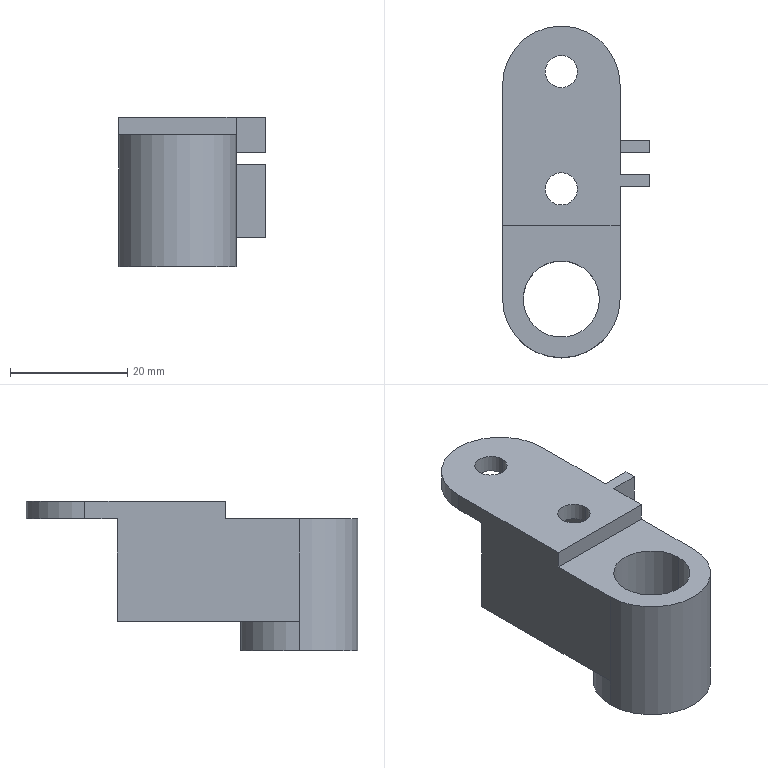Component | SolidWorks | CLS-MechanismAccessory1-1 | 1 solid | 31 faces | box 25 x 56.5 x 25.5 mm | volume 10042 mm3 | plane 21 | cylinder 10 | commonest cylinder face diameters 5.5 x4 20 x4 13 x2
STEP:
#1=COLOUR_RGB('',0.7922,0.8196,0.9333);
#2=FILL_AREA_STYLE_COLOUR('',#1);
#3=FILL_AREA_STYLE('',(#2));
#4=SURFACE_STYLE_FILL_AREA(#3);
#5=SURFACE_SIDE_STYLE('',(#4));
#6=SURFACE_STYLE_USAGE(.BOTH.,#5);
#7=PRESENTATION_STYLE_ASSIGNMENT((#6));
#8=CARTESIAN_POINT('',(-2.216,-0.1794,-0.1181));
#9=VERTEX_POINT('',#8);
#10=CARTESIAN_POINT('',(-2.432,-0.1794,-0.1181));
#11=VERTEX_POINT('',#10);
#12=CARTESIAN_POINT('',(-2.324,-0.1794,-0.1181));
#13=DIRECTION('',(-0.,0.,1.));
#14=DIRECTION('',(-1.,0.,0.));
#15=AXIS2_PLACEMENT_3D('',#12,#13,#14);
#16=CIRCLE('',#15,0.1083);
#17=EDGE_CURVE('',#9,#11,#16,.T.);
#18=ORIENTED_EDGE('',*,*,#17,.T.);
#19=CARTESIAN_POINT('',(-2.432,-0.1794,-0.2362));
#20=VERTEX_POINT('',#19);
#21=CARTESIAN_POINT('',(-2.432,-0.1794,-0.1181));
#22=DIRECTION('',(0.,-0.,-1.));
#23=VECTOR('',#22,39.37);
#24=LINE('',#21,#23);
#25=EDGE_CURVE('',#11,#20,#24,.T.);
#26=ORIENTED_EDGE('',*,*,#25,.T.);
#27=CARTESIAN_POINT('',(-2.216,-0.1794,-0.2362));
#28=VERTEX_POINT('',#27);
#29=CARTESIAN_POINT('',(-2.324,-0.1794,-0.2362));
#30=DIRECTION('',(0.,-0.,-1.));
#31=DIRECTION('',(1.,0.,0.));
#32=AXIS2_PLACEMENT_3D('',#29,#30,#31);
#33=CIRCLE('',#32,0.1083);
#34=EDGE_CURVE('',#20,#28,#33,.T.);
#35=ORIENTED_EDGE('',*,*,#34,.T.);
#36=CARTESIAN_POINT('',(-2.216,-0.1794,-0.1181));
#37=DIRECTION('',(0.,-0.,-1.));
#38=VECTOR('',#37,39.37);
#39=LINE('',#36,#38);
#40=EDGE_CURVE('',#9,#28,#39,.T.);
#41=ORIENTED_EDGE('',*,*,#40,.F.);
#42=EDGE_LOOP('',(#18,#26,#35,#41));
#43=FACE_OUTER_BOUND('',#42,.T.);
#44=CARTESIAN_POINT('',(-2.324,-0.1794,-0.1181));
#45=DIRECTION('',(0.,-0.,-1.));
#46=DIRECTION('',(1.,0.,0.));
#47=AXIS2_PLACEMENT_3D('',#44,#45,#46);
#48=CYLINDRICAL_SURFACE('',#47,0.1083);
#49=ADVANCED_FACE('',(#43),#48,.F.);
#50=CARTESIAN_POINT('',(-2.216,0.608,-0.1181));
#51=VERTEX_POINT('',#50);
#52=CARTESIAN_POINT('',(-2.432,0.608,-0.1181));
#53=VERTEX_POINT('',#52);
#54=CARTESIAN_POINT('',(-2.324,0.608,-0.1181));
#55=DIRECTION('',(-0.,0.,1.));
#56=DIRECTION('',(-1.,0.,0.));
#57=AXIS2_PLACEMENT_3D('',#54,#55,#56);
#58=CIRCLE('',#57,0.1083);
#59=EDGE_CURVE('',#51,#53,#58,.T.);
#60=ORIENTED_EDGE('',*,*,#59,.T.);
#61=CARTESIAN_POINT('',(-2.432,0.608,-0.2362));
#62=VERTEX_POINT('',#61);
#63=CARTESIAN_POINT('',(-2.432,0.608,-0.1181));
#64=DIRECTION('',(0.,-0.,-1.));
#65=VECTOR('',#64,39.37);
#66=LINE('',#63,#65);
#67=EDGE_CURVE('',#53,#62,#66,.T.);
#68=ORIENTED_EDGE('',*,*,#67,.T.);
#69=CARTESIAN_POINT('',(-2.216,0.608,-0.2362));
#70=VERTEX_POINT('',#69);
#71=CARTESIAN_POINT('',(-2.324,0.608,-0.2362));
#72=DIRECTION('',(0.,-0.,-1.));
#73=DIRECTION('',(1.,0.,0.));
#74=AXIS2_PLACEMENT_3D('',#71,#72,#73);
#75=CIRCLE('',#74,0.1083);
#76=EDGE_CURVE('',#62,#70,#75,.T.);
#77=ORIENTED_EDGE('',*,*,#76,.T.);
#78=CARTESIAN_POINT('',(-2.216,0.608,-0.1181));
#79=DIRECTION('',(0.,-0.,-1.));
#80=VECTOR('',#79,39.37);
#81=LINE('',#78,#80);
#82=EDGE_CURVE('',#51,#70,#81,.T.);
#83=ORIENTED_EDGE('',*,*,#82,.F.);
#84=EDGE_LOOP('',(#60,#68,#77,#83));
#85=FACE_OUTER_BOUND('',#84,.T.);
#86=CARTESIAN_POINT('',(-2.324,0.608,-0.1181));
#87=DIRECTION('',(0.,-0.,-1.));
#88=DIRECTION('',(1.,0.,0.));
#89=AXIS2_PLACEMENT_3D('',#86,#87,#88);
#90=CYLINDRICAL_SURFACE('',#89,0.1083);
#91=ADVANCED_FACE('',(#85),#90,.F.);
#92=CARTESIAN_POINT('',(-2.58,-0.9176,-0.2362));
#93=VERTEX_POINT('',#92);
#94=CARTESIAN_POINT('',(-2.068,-0.9176,-0.2362));
#95=VERTEX_POINT('',#94);
#96=CARTESIAN_POINT('',(-2.324,-0.9176,-0.2362));
#97=DIRECTION('',(0.,-0.,-1.));
#98=DIRECTION('',(1.,0.,0.));
#99=AXIS2_PLACEMENT_3D('',#96,#97,#98);
#100=CIRCLE('',#99,0.2559);
#101=EDGE_CURVE('',#93,#95,#100,.T.);
#102=ORIENTED_EDGE('',*,*,#101,.F.);
#103=CARTESIAN_POINT('',(-2.58,-0.9176,-1.122));
#104=VERTEX_POINT('',#103);
#105=CARTESIAN_POINT('',(-2.58,-0.9176,-0.2362));
#106=DIRECTION('',(0.,-0.,-1.));
#107=VECTOR('',#106,39.37);
#108=LINE('',#105,#107);
#109=EDGE_CURVE('',#93,#104,#108,.T.);
#110=ORIENTED_EDGE('',*,*,#109,.T.);
#111=CARTESIAN_POINT('',(-2.068,-0.9176,-1.122));
#112=VERTEX_POINT('',#111);
#113=CARTESIAN_POINT('',(-2.324,-0.9176,-1.122));
#114=DIRECTION('',(0.,-0.,-1.));
#115=DIRECTION('',(1.,0.,0.));
#116=AXIS2_PLACEMENT_3D('',#113,#114,#115);
#117=CIRCLE('',#116,0.2559);
#118=EDGE_CURVE('',#104,#112,#117,.T.);
#119=ORIENTED_EDGE('',*,*,#118,.T.);
#120=CARTESIAN_POINT('',(-2.068,-0.9176,-0.2362));
#121=DIRECTION('',(0.,-0.,-1.));
#122=VECTOR('',#121,39.37);
#123=LINE('',#120,#122);
#124=EDGE_CURVE('',#95,#112,#123,.T.);
#125=ORIENTED_EDGE('',*,*,#124,.F.);
#126=EDGE_LOOP('',(#102,#110,#119,#125));
#127=FACE_OUTER_BOUND('',#126,.T.);
#128=CARTESIAN_POINT('',(-2.324,-0.9176,-0.2362));
#129=DIRECTION('',(0.,-0.,-1.));
#130=DIRECTION('',(1.,0.,0.));
#131=AXIS2_PLACEMENT_3D('',#128,#129,#130);
#132=CYLINDRICAL_SURFACE('',#131,0.2559);
#133=ADVANCED_FACE('',(#127),#132,.F.);
#134=CARTESIAN_POINT('',(-1.93,-0.9176,-1.122));
#135=VERTEX_POINT('',#134);
#136=CARTESIAN_POINT('',(-2.718,-0.9176,-1.122));
#137=VERTEX_POINT('',#136);
#138=CARTESIAN_POINT('',(-2.324,-0.9176,-1.122));
#139=DIRECTION('',(0.,-0.,-1.));
#140=DIRECTION('',(1.,0.,0.));
#141=AXIS2_PLACEMENT_3D('',#138,#139,#140);
#142=CIRCLE('',#141,0.3937);
#143=EDGE_CURVE('',#135,#137,#142,.T.);
#144=ORIENTED_EDGE('',*,*,#143,.F.);
#145=CARTESIAN_POINT('',(-1.93,-0.9176,-0.9252));
#146=VERTEX_POINT('',#145);
#147=CARTESIAN_POINT('',(-1.93,-0.9176,-0.9252));
#148=DIRECTION('',(-0.,0.,1.));
#149=VECTOR('',#148,39.37);
#150=LINE('',#147,#149);
#151=EDGE_CURVE('',#135,#146,#150,.T.);
#152=ORIENTED_EDGE('',*,*,#151,.T.);
#153=CARTESIAN_POINT('',(-1.93,-0.9176,-0.2362));
#154=VERTEX_POINT('',#153);
#155=CARTESIAN_POINT('',(-1.93,-0.9176,-0.9252));
#156=DIRECTION('',(0.,-0.,-1.));
#157=VECTOR('',#156,39.37);
#158=LINE('',#155,#157);
#159=EDGE_CURVE('',#154,#146,#158,.T.);
#160=ORIENTED_EDGE('',*,*,#159,.F.);
#161=CARTESIAN_POINT('',(-2.718,-0.9176,-0.2362));
#162=VERTEX_POINT('',#161);
#163=CARTESIAN_POINT('',(-2.324,-0.9176,-0.2362));
#164=DIRECTION('',(-0.,0.,1.));
#165=DIRECTION('',(1.,0.,0.));
#166=AXIS2_PLACEMENT_3D('',#163,#164,#165);
#167=CIRCLE('',#166,0.3937);
#168=EDGE_CURVE('',#162,#154,#167,.T.);
#169=ORIENTED_EDGE('',*,*,#168,.F.);
#170=CARTESIAN_POINT('',(-2.718,-0.9176,-0.9252));
#171=VERTEX_POINT('',#170);
#172=CARTESIAN_POINT('',(-2.718,-0.9176,-0.9252));
#173=DIRECTION('',(-0.,0.,1.));
#174=VECTOR('',#173,39.37);
#175=LINE('',#172,#174);
#176=EDGE_CURVE('',#171,#162,#175,.T.);
#177=ORIENTED_EDGE('',*,*,#176,.F.);
#178=CARTESIAN_POINT('',(-2.718,-0.9176,-0.9252));
#179=DIRECTION('',(-0.,0.,1.));
#180=VECTOR('',#179,39.37);
#181=LINE('',#178,#180);
#182=EDGE_CURVE('',#137,#171,#181,.T.);
#183=ORIENTED_EDGE('',*,*,#182,.F.);
#184=EDGE_LOOP('',(#144,#152,#160,#169,#177,#183));
#185=FACE_OUTER_BOUND('',#184,.T.);
#186=CARTESIAN_POINT('',(-2.324,-0.9176,-0.9252));
#187=DIRECTION('',(-0.,0.,1.));
#188=DIRECTION('',(-1.,0.,0.));
#189=AXIS2_PLACEMENT_3D('',#186,#187,#188);
#190=CYLINDRICAL_SURFACE('',#189,0.3937);
#191=ADVANCED_FACE('',(#185),#190,.T.);
#192=CARTESIAN_POINT('',(-1.93,-0.1614,-0.1181));
#193=VERTEX_POINT('',#192);
#194=CARTESIAN_POINT('',(-1.93,-0.1614,-0.3544));
#195=VERTEX_POINT('',#194);
#196=CARTESIAN_POINT('',(-1.93,-0.1614,-0.1181));
#197=DIRECTION('',(0.,-0.,-1.));
#198=VECTOR('',#197,39.37);
#199=LINE('',#196,#198);
#200=EDGE_CURVE('',#193,#195,#199,.T.);
#201=ORIENTED_EDGE('',*,*,#200,.F.);
#202=CARTESIAN_POINT('',(-1.93,-0.4255,-0.1181));
#203=VERTEX_POINT('',#202);
#204=CARTESIAN_POINT('',(-1.93,-0.4255,-0.1181));
#205=DIRECTION('',(-0.,1.,-0.));
#206=VECTOR('',#205,39.37);
#207=LINE('',#204,#206);
#208=EDGE_CURVE('',#203,#193,#207,.T.);
#209=ORIENTED_EDGE('',*,*,#208,.F.);
#210=CARTESIAN_POINT('',(-1.93,-0.4255,-0.2362));
#211=VERTEX_POINT('',#210);
#212=CARTESIAN_POINT('',(-1.93,-0.4255,-0.1181));
#213=DIRECTION('',(0.,-0.,-1.));
#214=VECTOR('',#213,39.37);
#215=LINE('',#212,#214);
#216=EDGE_CURVE('',#203,#211,#215,.T.);
#217=ORIENTED_EDGE('',*,*,#216,.T.);
#218=CARTESIAN_POINT('',(-1.93,-1.311,-0.2362));
#219=DIRECTION('',(-0.,-1.,0.));
#220=VECTOR('',#219,39.37);
#221=LINE('',#218,#220);
#222=EDGE_CURVE('',#211,#154,#221,.T.);
#223=ORIENTED_EDGE('',*,*,#222,.T.);
#224=ORIENTED_EDGE('',*,*,#159,.T.);
#225=CARTESIAN_POINT('',(-1.93,0.06662,-0.9252));
#226=VERTEX_POINT('',#225);
#227=CARTESIAN_POINT('',(-1.93,-1.311,-0.9252));
#228=DIRECTION('',(-0.,-1.,0.));
#229=VECTOR('',#228,39.37);
#230=LINE('',#227,#229);
#231=EDGE_CURVE('',#226,#146,#230,.T.);
#232=ORIENTED_EDGE('',*,*,#231,.F.);
#233=CARTESIAN_POINT('',(-1.93,0.06662,-0.4331));
#234=VERTEX_POINT('',#233);
#235=CARTESIAN_POINT('',(-1.93,0.06662,-0.9252));
#236=DIRECTION('',(0.,-0.,-1.));
#237=VECTOR('',#236,39.37);
#238=LINE('',#235,#237);
#239=EDGE_CURVE('',#234,#226,#238,.T.);
#240=ORIENTED_EDGE('',*,*,#239,.F.);
#241=CARTESIAN_POINT('',(-1.93,0.1454,-0.4331));
#242=VERTEX_POINT('',#241);
#243=CARTESIAN_POINT('',(-1.93,0.06662,-0.4331));
#244=DIRECTION('',(-0.,-1.,0.));
#245=VECTOR('',#244,39.37);
#246=LINE('',#243,#245);
#247=EDGE_CURVE('',#242,#234,#246,.T.);
#248=ORIENTED_EDGE('',*,*,#247,.F.);
#249=CARTESIAN_POINT('',(-1.93,0.1454,-0.9252));
#250=VERTEX_POINT('',#249);
#251=CARTESIAN_POINT('',(-1.93,0.1454,-0.9252));
#252=DIRECTION('',(-0.,0.,1.));
#253=VECTOR('',#252,39.37);
#254=LINE('',#251,#253);
#255=EDGE_CURVE('',#250,#242,#254,.T.);
#256=ORIENTED_EDGE('',*,*,#255,.F.);
#257=CARTESIAN_POINT('',(-1.93,0.3028,-0.9252));
#258=VERTEX_POINT('',#257);
#259=CARTESIAN_POINT('',(-1.93,-1.311,-0.9252));
#260=DIRECTION('',(-0.,-1.,0.));
#261=VECTOR('',#260,39.37);
#262=LINE('',#259,#261);
#263=EDGE_CURVE('',#258,#250,#262,.T.);
#264=ORIENTED_EDGE('',*,*,#263,.F.);
#265=CARTESIAN_POINT('',(-1.93,0.3028,-0.2362));
#266=VERTEX_POINT('',#265);
#267=CARTESIAN_POINT('',(-1.93,0.3028,-0.9252));
#268=DIRECTION('',(-0.,0.,1.));
#269=VECTOR('',#268,39.37);
#270=LINE('',#267,#269);
#271=EDGE_CURVE('',#258,#266,#270,.T.);
#272=ORIENTED_EDGE('',*,*,#271,.T.);
#273=CARTESIAN_POINT('',(-1.93,0.5194,-0.2362));
#274=VERTEX_POINT('',#273);
#275=CARTESIAN_POINT('',(-1.93,-0.4255,-0.2362));
#276=DIRECTION('',(-0.,1.,-0.));
#277=VECTOR('',#276,39.37);
#278=LINE('',#275,#277);
#279=EDGE_CURVE('',#266,#274,#278,.T.);
#280=ORIENTED_EDGE('',*,*,#279,.T.);
#281=CARTESIAN_POINT('',(-1.93,0.5194,-0.1181));
#282=VERTEX_POINT('',#281);
#283=CARTESIAN_POINT('',(-1.93,0.5194,-0.9252));
#284=DIRECTION('',(-0.,0.,1.));
#285=VECTOR('',#284,39.37);
#286=LINE('',#283,#285);
#287=EDGE_CURVE('',#274,#282,#286,.T.);
#288=ORIENTED_EDGE('',*,*,#287,.T.);
#289=CARTESIAN_POINT('',(-1.93,-0.08265,-0.1181));
#290=VERTEX_POINT('',#289);
#291=CARTESIAN_POINT('',(-1.93,-0.4255,-0.1181));
#292=DIRECTION('',(-0.,1.,-0.));
#293=VECTOR('',#292,39.37);
#294=LINE('',#291,#293);
#295=EDGE_CURVE('',#290,#282,#294,.T.);
#296=ORIENTED_EDGE('',*,*,#295,.F.);
#297=CARTESIAN_POINT('',(-1.93,-0.08265,-0.3544));
#298=VERTEX_POINT('',#297);
#299=CARTESIAN_POINT('',(-1.93,-0.08265,-0.1181));
#300=DIRECTION('',(-0.,0.,1.));
#301=VECTOR('',#300,39.37);
#302=LINE('',#299,#301);
#303=EDGE_CURVE('',#298,#290,#302,.T.);
#304=ORIENTED_EDGE('',*,*,#303,.F.);
#305=CARTESIAN_POINT('',(-1.93,-0.08265,-0.3544));
#306=DIRECTION('',(-0.,1.,-0.));
#307=VECTOR('',#306,39.37);
#308=LINE('',#305,#307);
#309=EDGE_CURVE('',#195,#298,#308,.T.);
#310=ORIENTED_EDGE('',*,*,#309,.F.);
#311=EDGE_LOOP('',(#201,#209,#217,#223,#224,#232,#240,#248,#256,#264,#272,#280,#288,#296,#304,#310));
#312=FACE_OUTER_BOUND('',#311,.T.);
#313=CARTESIAN_POINT('',(-1.93,-1.311,-0.9252));
#314=DIRECTION('',(-1.,0.,-0.));
#315=DIRECTION('',(0.,1.,-0.));
#316=AXIS2_PLACEMENT_3D('',#313,#314,#315);
#317=PLANE('',#316);
#318=ADVANCED_FACE('',(#312),#317,.F.);
#319=CARTESIAN_POINT('',(-2.324,-0.9176,-0.2362));
#320=DIRECTION('',(0.,-0.,-1.));
#321=DIRECTION('',(1.,0.,0.));
#322=AXIS2_PLACEMENT_3D('',#319,#320,#321);
#323=CIRCLE('',#322,0.2559);
#324=EDGE_CURVE('',#95,#93,#323,.T.);
#325=ORIENTED_EDGE('',*,*,#324,.T.);
#326=ORIENTED_EDGE('',*,*,#101,.T.);
#327=EDGE_LOOP('',(#325,#326));
#328=FACE_BOUND('',#327,.T.);
#329=CARTESIAN_POINT('',(-2.718,-0.4255,-0.2362));
#330=VERTEX_POINT('',#329);
#331=CARTESIAN_POINT('',(-1.93,-0.4255,-0.2362));
#332=DIRECTION('',(1.,0.,0.));
#333=VECTOR('',#332,39.37);
#334=LINE('',#331,#333);
#335=EDGE_CURVE('',#330,#211,#334,.T.);
#336=ORIENTED_EDGE('',*,*,#335,.F.);
#337=CARTESIAN_POINT('',(-2.718,-1.311,-0.2362));
#338=DIRECTION('',(-0.,1.,-0.));
#339=VECTOR('',#338,39.37);
#340=LINE('',#337,#339);
#341=EDGE_CURVE('',#162,#330,#340,.T.);
#342=ORIENTED_EDGE('',*,*,#341,.F.);
#343=ORIENTED_EDGE('',*,*,#168,.T.);
#344=ORIENTED_EDGE('',*,*,#222,.F.);
#345=EDGE_LOOP('',(#336,#342,#343,#344));
#346=FACE_OUTER_BOUND('',#345,.T.);
#347=CARTESIAN_POINT('',(-1.93,0.3028,-0.2362));
#348=DIRECTION('',(0.,-0.,-1.));
#349=DIRECTION('',(1.,0.,0.));
#350=AXIS2_PLACEMENT_3D('',#347,#348,#349);
#351=PLANE('',#350);
#352=ADVANCED_FACE('',(#328,#346),#351,.F.);
#353=CARTESIAN_POINT('',(-2.068,0.3028,-0.9252));
#354=VERTEX_POINT('',#353);
#355=CARTESIAN_POINT('',(-2.718,0.3028,-0.9252));
#356=DIRECTION('',(1.,0.,0.));
#357=VECTOR('',#356,39.37);
#358=LINE('',#355,#357);
#359=EDGE_CURVE('',#354,#258,#358,.T.);
#360=ORIENTED_EDGE('',*,*,#359,.F.);
#361=CARTESIAN_POINT('',(-2.068,0.3028,-0.2362));
#362=VERTEX_POINT('',#361);
#363=CARTESIAN_POINT('',(-2.068,0.3028,-0.9252));
#364=DIRECTION('',(-0.,0.,1.));
#365=VECTOR('',#364,39.37);
#366=LINE('',#363,#365);
#367=EDGE_CURVE('',#354,#362,#366,.T.);
#368=ORIENTED_EDGE('',*,*,#367,.T.);
#369=CARTESIAN_POINT('',(-2.718,0.3028,-0.2362));
#370=DIRECTION('',(1.,0.,0.));
#371=VECTOR('',#370,39.37);
#372=LINE('',#369,#371);
#373=EDGE_CURVE('',#362,#266,#372,.T.);
#374=ORIENTED_EDGE('',*,*,#373,.T.);
#375=ORIENTED_EDGE('',*,*,#271,.F.);
#376=EDGE_LOOP('',(#360,#368,#374,#375));
#377=FACE_OUTER_BOUND('',#376,.T.);
#378=CARTESIAN_POINT('',(-2.718,0.3028,-0.9252));
#379=DIRECTION('',(0.,-1.,0.));
#380=DIRECTION('',(0.,-0.,-1.));
#381=AXIS2_PLACEMENT_3D('',#378,#379,#380);
#382=PLANE('',#381);
#383=ADVANCED_FACE('',(#377),#382,.F.);
#384=CARTESIAN_POINT('',(-2.718,0.5194,-0.1181));
#385=VERTEX_POINT('',#384);
#386=CARTESIAN_POINT('',(-2.718,-0.4255,-0.1181));
#387=VERTEX_POINT('',#386);
#388=CARTESIAN_POINT('',(-2.718,-0.4255,-0.1181));
#389=DIRECTION('',(0.,-1.,0.));
#390=VECTOR('',#389,39.37);
#391=LINE('',#388,#390);
#392=EDGE_CURVE('',#385,#387,#391,.T.);
#393=ORIENTED_EDGE('',*,*,#392,.F.);
#394=CARTESIAN_POINT('',(-2.718,0.5194,-0.2362));
#395=VERTEX_POINT('',#394);
#396=CARTESIAN_POINT('',(-2.718,0.5194,-0.9252));
#397=DIRECTION('',(0.,-0.,-1.));
#398=VECTOR('',#397,39.37);
#399=LINE('',#396,#398);
#400=EDGE_CURVE('',#385,#395,#399,.T.);
#401=ORIENTED_EDGE('',*,*,#400,.T.);
#402=CARTESIAN_POINT('',(-2.718,0.3028,-0.2362));
#403=VERTEX_POINT('',#402);
#404=CARTESIAN_POINT('',(-2.718,-0.4255,-0.2362));
#405=DIRECTION('',(0.,-1.,0.));
#406=VECTOR('',#405,39.37);
#407=LINE('',#404,#406);
#408=EDGE_CURVE('',#395,#403,#407,.T.);
#409=ORIENTED_EDGE('',*,*,#408,.T.);
#410=CARTESIAN_POINT('',(-2.718,0.3028,-0.9252));
#411=VERTEX_POINT('',#410);
#412=CARTESIAN_POINT('',(-2.718,0.3028,-0.9252));
#413=DIRECTION('',(-0.,0.,1.));
#414=VECTOR('',#413,39.37);
#415=LINE('',#412,#414);
#416=EDGE_CURVE('',#411,#403,#415,.T.);
#417=ORIENTED_EDGE('',*,*,#416,.F.);
#418=CARTESIAN_POINT('',(-2.718,-1.311,-0.9252));
#419=DIRECTION('',(-0.,1.,-0.));
#420=VECTOR('',#419,39.37);
#421=LINE('',#418,#420);
#422=EDGE_CURVE('',#171,#411,#421,.T.);
#423=ORIENTED_EDGE('',*,*,#422,.F.);
#424=ORIENTED_EDGE('',*,*,#176,.T.);
#425=ORIENTED_EDGE('',*,*,#341,.T.);
#426=CARTESIAN_POINT('',(-2.718,-0.4255,-0.1181));
#427=DIRECTION('',(0.,-0.,-1.));
#428=VECTOR('',#427,39.37);
#429=LINE('',#426,#428);
#430=EDGE_CURVE('',#387,#330,#429,.T.);
#431=ORIENTED_EDGE('',*,*,#430,.F.);
#432=EDGE_LOOP('',(#393,#401,#409,#417,#423,#424,#425,#431));
#433=FACE_OUTER_BOUND('',#432,.T.);
#434=CARTESIAN_POINT('',(-2.718,-1.311,-0.9252));
#435=DIRECTION('',(1.,0.,0.));
#436=DIRECTION('',(0.,-1.,0.));
#437=AXIS2_PLACEMENT_3D('',#434,#435,#436);
#438=PLANE('',#437);
#439=ADVANCED_FACE('',(#433),#438,.F.);
#440=CARTESIAN_POINT('',(-2.58,0.3028,-0.2362));
#441=VERTEX_POINT('',#440);
#442=CARTESIAN_POINT('',(-2.718,0.3028,-0.2362));
#443=DIRECTION('',(1.,0.,0.));
#444=VECTOR('',#443,39.37);
#445=LINE('',#442,#444);
#446=EDGE_CURVE('',#403,#441,#445,.T.);
#447=ORIENTED_EDGE('',*,*,#446,.T.);
#448=CARTESIAN_POINT('',(-2.58,0.3028,-0.9252));
#449=VERTEX_POINT('',#448);
#450=CARTESIAN_POINT('',(-2.58,0.3028,-0.9252));
#451=DIRECTION('',(0.,-0.,-1.));
#452=VECTOR('',#451,39.37);
#453=LINE('',#450,#452);
#454=EDGE_CURVE('',#441,#449,#453,.T.);
#455=ORIENTED_EDGE('',*,*,#454,.T.);
#456=CARTESIAN_POINT('',(-2.718,0.3028,-0.9252));
#457=DIRECTION('',(1.,0.,0.));
#458=VECTOR('',#457,39.37);
#459=LINE('',#456,#458);
#460=EDGE_CURVE('',#411,#449,#459,.T.);
#461=ORIENTED_EDGE('',*,*,#460,.F.);
#462=ORIENTED_EDGE('',*,*,#416,.T.);
#463=EDGE_LOOP('',(#447,#455,#461,#462));
#464=FACE_OUTER_BOUND('',#463,.T.);
#465=CARTESIAN_POINT('',(-2.718,0.3028,-0.9252));
#466=DIRECTION('',(0.,-1.,0.));
#467=DIRECTION('',(0.,-0.,-1.));
#468=AXIS2_PLACEMENT_3D('',#465,#466,#467);
#469=PLANE('',#468);
#470=ADVANCED_FACE('',(#464),#469,.F.);
#471=CARTESIAN_POINT('',(-2.068,-0.4058,-0.9252));
#472=VERTEX_POINT('',#471);
#473=CARTESIAN_POINT('',(-2.068,1.011,-0.9252));
#474=DIRECTION('',(0.,-1.,0.));
#475=VECTOR('',#474,39.37);
#476=LINE('',#473,#475);
#477=EDGE_CURVE('',#354,#472,#476,.T.);
#478=ORIENTED_EDGE('',*,*,#477,.F.);
#479=ORIENTED_EDGE('',*,*,#359,.T.);
#480=ORIENTED_EDGE('',*,*,#263,.T.);
#481=CARTESIAN_POINT('',(-1.733,0.1454,-0.9252));
#482=VERTEX_POINT('',#481);
#483=CARTESIAN_POINT('',(-1.733,0.1454,-0.9252));
#484=DIRECTION('',(-1.,0.,-0.));
#485=VECTOR('',#484,39.37);
#486=LINE('',#483,#485);
#487=EDGE_CURVE('',#482,#250,#486,.T.);
#488=ORIENTED_EDGE('',*,*,#487,.F.);
#489=CARTESIAN_POINT('',(-1.733,0.06662,-0.9252));
#490=VERTEX_POINT('',#489);
#491=CARTESIAN_POINT('',(-1.733,0.06662,-0.9252));
#492=DIRECTION('',(0.,1.,-0.));
#493=VECTOR('',#492,39.37);
#494=LINE('',#491,#493);
#495=EDGE_CURVE('',#490,#482,#494,.T.);
#496=ORIENTED_EDGE('',*,*,#495,.F.);
#497=CARTESIAN_POINT('',(-1.733,0.06662,-0.9252));
#498=DIRECTION('',(-1.,0.,-0.));
#499=VECTOR('',#498,39.37);
#500=LINE('',#497,#499);
#501=EDGE_CURVE('',#490,#226,#500,.T.);
#502=ORIENTED_EDGE('',*,*,#501,.T.);
#503=ORIENTED_EDGE('',*,*,#231,.T.);
#504=CARTESIAN_POINT('',(-2.324,-0.9176,-0.9252));
#505=DIRECTION('',(0.,-0.,-1.));
#506=DIRECTION('',(1.,0.,0.));
#507=AXIS2_PLACEMENT_3D('',#504,#505,#506);
#508=CIRCLE('',#507,0.3937);
#509=EDGE_CURVE('',#171,#146,#508,.T.);
#510=ORIENTED_EDGE('',*,*,#509,.F.);
#511=ORIENTED_EDGE('',*,*,#422,.T.);
#512=ORIENTED_EDGE('',*,*,#460,.T.);
#513=CARTESIAN_POINT('',(-2.58,-0.4058,-0.9252));
#514=VERTEX_POINT('',#513);
#515=CARTESIAN_POINT('',(-2.58,1.011,-0.9252));
#516=DIRECTION('',(-0.,1.,-0.));
#517=VECTOR('',#516,39.37);
#518=LINE('',#515,#517);
#519=EDGE_CURVE('',#514,#449,#518,.T.);
#520=ORIENTED_EDGE('',*,*,#519,.F.);
#521=CARTESIAN_POINT('',(-2.58,-0.4058,-0.9252));
#522=DIRECTION('',(-1.,-0.,-0.));
#523=VECTOR('',#522,39.37);
#524=LINE('',#521,#523);
#525=EDGE_CURVE('',#472,#514,#524,.T.);
#526=ORIENTED_EDGE('',*,*,#525,.F.);
#527=EDGE_LOOP('',(#478,#479,#480,#488,#496,#502,#503,#510,#511,#512,#520,#526));
#528=FACE_OUTER_BOUND('',#527,.T.);
#529=CARTESIAN_POINT('',(-1.93,0.3028,-0.9252));
#530=DIRECTION('',(0.,-0.,-1.));
#531=DIRECTION('',(1.,0.,0.));
#532=AXIS2_PLACEMENT_3D('',#529,#530,#531);
#533=PLANE('',#532);
#534=ADVANCED_FACE('',(#528),#533,.T.);
#535=ORIENTED_EDGE('',*,*,#151,.F.);
#536=CARTESIAN_POINT('',(-2.324,-0.9176,-1.122));
#537=DIRECTION('',(0.,-0.,-1.));
#538=DIRECTION('',(1.,0.,0.));
#539=AXIS2_PLACEMENT_3D('',#536,#537,#538);
#540=CIRCLE('',#539,0.3937);
#541=EDGE_CURVE('',#137,#135,#540,.T.);
#542=ORIENTED_EDGE('',*,*,#541,.F.);
#543=ORIENTED_EDGE('',*,*,#182,.T.);
#544=ORIENTED_EDGE('',*,*,#509,.T.);
#545=EDGE_LOOP('',(#535,#542,#543,#544));
#546=FACE_OUTER_BOUND('',#545,.T.);
#547=CARTESIAN_POINT('',(-2.324,-0.9176,-0.9252));
#548=DIRECTION('',(-0.,0.,1.));
#549=DIRECTION('',(-1.,0.,0.));
#550=AXIS2_PLACEMENT_3D('',#547,#548,#549);
#551=CYLINDRICAL_SURFACE('',#550,0.3937);
#552=ADVANCED_FACE('',(#546),#551,.T.);
#553=ORIENTED_EDGE('',*,*,#109,.F.);
#554=ORIENTED_EDGE('',*,*,#324,.F.);
#555=ORIENTED_EDGE('',*,*,#124,.T.);
#556=CARTESIAN_POINT('',(-2.324,-0.9176,-1.122));
#557=DIRECTION('',(0.,-0.,-1.));
#558=DIRECTION('',(1.,0.,0.));
#559=AXIS2_PLACEMENT_3D('',#556,#557,#558);
#560=CIRCLE('',#559,0.2559);
#561=EDGE_CURVE('',#112,#104,#560,.T.);
#562=ORIENTED_EDGE('',*,*,#561,.T.);
#563=EDGE_LOOP('',(#553,#554,#555,#562));
#564=FACE_OUTER_BOUND('',#563,.T.);
#565=CARTESIAN_POINT('',(-2.324,-0.9176,-0.2362));
#566=DIRECTION('',(0.,-0.,-1.));
#567=DIRECTION('',(1.,0.,0.));
#568=AXIS2_PLACEMENT_3D('',#565,#566,#567);
#569=CYLINDRICAL_SURFACE('',#568,0.2559);
#570=ADVANCED_FACE('',(#564),#569,.F.);
#571=ORIENTED_EDGE('',*,*,#541,.T.);
#572=ORIENTED_EDGE('',*,*,#143,.T.);
#573=EDGE_LOOP('',(#571,#572));
#574=FACE_OUTER_BOUND('',#573,.T.);
#575=ORIENTED_EDGE('',*,*,#561,.F.);
#576=ORIENTED_EDGE('',*,*,#118,.F.);
#577=EDGE_LOOP('',(#575,#576));
#578=FACE_BOUND('',#577,.T.);
#579=CARTESIAN_POINT('',(-2.324,-0.9176,-1.122));
#580=DIRECTION('',(0.,-0.,-1.));
#581=DIRECTION('',(1.,0.,0.));
#582=AXIS2_PLACEMENT_3D('',#579,#580,#581);
#583=PLANE('',#582);
#584=ADVANCED_FACE('',(#574,#578),#583,.T.);
#585=ORIENTED_EDGE('',*,*,#477,.T.);
#586=CARTESIAN_POINT('',(-2.068,-0.4058,-0.2362));
#587=VERTEX_POINT('',#586);
#588=CARTESIAN_POINT('',(-2.068,-0.4058,-0.2362));
#589=DIRECTION('',(0.,-0.,-1.));
#590=VECTOR('',#589,39.37);
#591=LINE('',#588,#590);
#592=EDGE_CURVE('',#587,#472,#591,.T.);
#593=ORIENTED_EDGE('',*,*,#592,.F.);
#594=CARTESIAN_POINT('',(-2.068,0.3028,-0.2362));
#595=DIRECTION('',(0.,-1.,0.));
#596=VECTOR('',#595,39.37);
#597=LINE('',#594,#596);
#598=EDGE_CURVE('',#362,#587,#597,.T.);
#599=ORIENTED_EDGE('',*,*,#598,.F.);
#600=ORIENTED_EDGE('',*,*,#367,.F.);
#601=EDGE_LOOP('',(#585,#593,#599,#600));
#602=FACE_OUTER_BOUND('',#601,.T.);
#603=CARTESIAN_POINT('',(-2.068,1.011,-0.2362));
#604=DIRECTION('',(1.,0.,0.));
#605=DIRECTION('',(0.,-1.,0.));
#606=AXIS2_PLACEMENT_3D('',#603,#604,#605);
#607=PLANE('',#606);
#608=ADVANCED_FACE('',(#602),#607,.F.);
#609=CARTESIAN_POINT('',(-2.58,-0.4058,-0.2362));
#610=VERTEX_POINT('',#609);
#611=CARTESIAN_POINT('',(-2.58,0.3028,-0.2362));
#612=DIRECTION('',(-0.,1.,-0.));
#613=VECTOR('',#612,39.37);
#614=LINE('',#611,#613);
#615=EDGE_CURVE('',#610,#441,#614,.T.);
#616=ORIENTED_EDGE('',*,*,#615,.F.);
#617=CARTESIAN_POINT('',(-2.58,-0.4058,-0.2362));
#618=DIRECTION('',(0.,-0.,-1.));
#619=VECTOR('',#618,39.37);
#620=LINE('',#617,#619);
#621=EDGE_CURVE('',#610,#514,#620,.T.);
#622=ORIENTED_EDGE('',*,*,#621,.T.);
#623=ORIENTED_EDGE('',*,*,#519,.T.);
#624=ORIENTED_EDGE('',*,*,#454,.F.);
#625=EDGE_LOOP('',(#616,#622,#623,#624));
#626=FACE_OUTER_BOUND('',#625,.T.);
#627=CARTESIAN_POINT('',(-2.58,1.011,-0.2362));
#628=DIRECTION('',(-1.,-0.,-0.));
#629=DIRECTION('',(-0.,1.,-0.));
#630=AXIS2_PLACEMENT_3D('',#627,#628,#629);
#631=PLANE('',#630);
#632=ADVANCED_FACE('',(#626),#631,.F.);
#633=ORIENTED_EDGE('',*,*,#592,.T.);
#634=ORIENTED_EDGE('',*,*,#525,.T.);
#635=ORIENTED_EDGE('',*,*,#621,.F.);
#636=CARTESIAN_POINT('',(-1.93,-0.4058,-0.2362));
#637=DIRECTION('',(-1.,-0.,-0.));
#638=VECTOR('',#637,39.37);
#639=LINE('',#636,#638);
#640=EDGE_CURVE('',#587,#610,#639,.T.);
#641=ORIENTED_EDGE('',*,*,#640,.F.);
#642=EDGE_LOOP('',(#633,#634,#635,#641));
#643=FACE_OUTER_BOUND('',#642,.T.);
#644=CARTESIAN_POINT('',(-2.58,-0.4058,-0.2362));
#645=DIRECTION('',(0.,-1.,0.));
#646=DIRECTION('',(-1.,-0.,-0.));
#647=AXIS2_PLACEMENT_3D('',#644,#645,#646);
#648=PLANE('',#647);
#649=ADVANCED_FACE('',(#643),#648,.F.);
#650=ORIENTED_EDGE('',*,*,#335,.T.);
#651=ORIENTED_EDGE('',*,*,#216,.F.);
#652=CARTESIAN_POINT('',(-1.93,-0.4255,-0.1181));
#653=DIRECTION('',(1.,0.,0.));
#654=VECTOR('',#653,39.37);
#655=LINE('',#652,#654);
#656=EDGE_CURVE('',#387,#203,#655,.T.);
#657=ORIENTED_EDGE('',*,*,#656,.F.);
#658=ORIENTED_EDGE('',*,*,#430,.T.);
#659=EDGE_LOOP('',(#650,#651,#657,#658));
#660=FACE_OUTER_BOUND('',#659,.T.);
#661=CARTESIAN_POINT('',(-1.93,-0.4255,-0.1181));
#662=DIRECTION('',(-0.,1.,-0.));
#663=DIRECTION('',(-0.,0.,1.));
#664=AXIS2_PLACEMENT_3D('',#661,#662,#663);
#665=PLANE('',#664);
#666=ADVANCED_FACE('',(#660),#665,.F.);
#667=ORIENTED_EDGE('',*,*,#17,.F.);
#668=CARTESIAN_POINT('',(-2.324,-0.1794,-0.1181));
#669=DIRECTION('',(-0.,0.,1.));
#670=DIRECTION('',(-1.,0.,0.));
#671=AXIS2_PLACEMENT_3D('',#668,#669,#670);
#672=CIRCLE('',#671,0.1083);
#673=EDGE_CURVE('',#11,#9,#672,.T.);
#674=ORIENTED_EDGE('',*,*,#673,.F.);
#675=EDGE_LOOP('',(#667,#674));
#676=FACE_BOUND('',#675,.T.);
#677=ORIENTED_EDGE('',*,*,#59,.F.);
#678=CARTESIAN_POINT('',(-2.324,0.608,-0.1181));
#679=DIRECTION('',(-0.,0.,1.));
#680=DIRECTION('',(-1.,0.,0.));
#681=AXIS2_PLACEMENT_3D('',#678,#679,#680);
#682=CIRCLE('',#681,0.1083);
#683=EDGE_CURVE('',#53,#51,#682,.T.);
#684=ORIENTED_EDGE('',*,*,#683,.F.);
#685=EDGE_LOOP('',(#677,#684));
#686=FACE_BOUND('',#685,.T.);
#687=ORIENTED_EDGE('',*,*,#208,.T.);
#688=CARTESIAN_POINT('',(-1.733,-0.1614,-0.1181));
#689=VERTEX_POINT('',#688);
#690=CARTESIAN_POINT('',(-1.733,-0.1614,-0.1181));
#691=DIRECTION('',(-1.,0.,-0.));
#692=VECTOR('',#691,39.37);
#693=LINE('',#690,#692);
#694=EDGE_CURVE('',#689,#193,#693,.T.);
#695=ORIENTED_EDGE('',*,*,#694,.F.);
#696=CARTESIAN_POINT('',(-1.733,-0.08265,-0.1181));
#697=VERTEX_POINT('',#696);
#698=CARTESIAN_POINT('',(-1.733,-0.08265,-0.1181));
#699=DIRECTION('',(0.,-1.,0.));
#700=VECTOR('',#699,39.37);
#701=LINE('',#698,#700);
#702=EDGE_CURVE('',#697,#689,#701,.T.);
#703=ORIENTED_EDGE('',*,*,#702,.F.);
#704=CARTESIAN_POINT('',(-1.733,-0.08265,-0.1181));
#705=DIRECTION('',(-1.,0.,-0.));
#706=VECTOR('',#705,39.37);
#707=LINE('',#704,#706);
#708=EDGE_CURVE('',#697,#290,#707,.T.);
#709=ORIENTED_EDGE('',*,*,#708,.T.);
#710=ORIENTED_EDGE('',*,*,#295,.T.);
#711=CARTESIAN_POINT('',(-2.324,0.9131,-0.1181));
#712=VERTEX_POINT('',#711);
#713=CARTESIAN_POINT('',(-2.324,0.5194,-0.1181));
#714=DIRECTION('',(-0.,0.,1.));
#715=DIRECTION('',(-1.,-0.,-0.));
#716=AXIS2_PLACEMENT_3D('',#713,#714,#715);
#717=CIRCLE('',#716,0.3937);
#718=EDGE_CURVE('',#282,#712,#717,.T.);
#719=ORIENTED_EDGE('',*,*,#718,.T.);
#720=CARTESIAN_POINT('',(-2.324,0.5194,-0.1181));
#721=DIRECTION('',(-0.,0.,1.));
#722=DIRECTION('',(-1.,-0.,-0.));
#723=AXIS2_PLACEMENT_3D('',#720,#721,#722);
#724=CIRCLE('',#723,0.3937);
#725=EDGE_CURVE('',#712,#385,#724,.T.);
#726=ORIENTED_EDGE('',*,*,#725,.T.);
#727=ORIENTED_EDGE('',*,*,#392,.T.);
#728=ORIENTED_EDGE('',*,*,#656,.T.);
#729=EDGE_LOOP('',(#687,#695,#703,#709,#710,#719,#726,#727,#728));
#730=FACE_OUTER_BOUND('',#729,.T.);
#731=CARTESIAN_POINT('',(-2.718,0.9131,-0.1181));
#732=DIRECTION('',(-0.,0.,1.));
#733=DIRECTION('',(-1.,-0.,-0.));
#734=AXIS2_PLACEMENT_3D('',#731,#732,#733);
#735=PLANE('',#734);
#736=ADVANCED_FACE('',(#676,#686,#730),#735,.T.);
#737=CARTESIAN_POINT('',(-2.324,-0.1794,-0.2362));
#738=DIRECTION('',(0.,-0.,-1.));
#739=DIRECTION('',(1.,0.,0.));
#740=AXIS2_PLACEMENT_3D('',#737,#738,#739);
#741=CIRCLE('',#740,0.1083);
#742=EDGE_CURVE('',#28,#20,#741,.T.);
#743=ORIENTED_EDGE('',*,*,#742,.F.);
#744=ORIENTED_EDGE('',*,*,#34,.F.);
#745=EDGE_LOOP('',(#743,#744));
#746=FACE_BOUND('',#745,.T.);
#747=CARTESIAN_POINT('',(-2.324,0.608,-0.2362));
#748=DIRECTION('',(0.,-0.,-1.));
#749=DIRECTION('',(1.,0.,0.));
#750=AXIS2_PLACEMENT_3D('',#747,#748,#749);
#751=CIRCLE('',#750,0.1083);
#752=EDGE_CURVE('',#70,#62,#751,.T.);
#753=ORIENTED_EDGE('',*,*,#752,.F.);
#754=ORIENTED_EDGE('',*,*,#76,.F.);
#755=EDGE_LOOP('',(#753,#754));
#756=FACE_BOUND('',#755,.T.);
#757=CARTESIAN_POINT('',(-2.324,0.9131,-0.2362));
#758=VERTEX_POINT('',#757);
#759=CARTESIAN_POINT('',(-2.324,0.5194,-0.2362));
#760=DIRECTION('',(0.,-0.,-1.));
#761=DIRECTION('',(-1.,-0.,0.));
#762=AXIS2_PLACEMENT_3D('',#759,#760,#761);
#763=CIRCLE('',#762,0.3937);
#764=EDGE_CURVE('',#395,#758,#763,.T.);
#765=ORIENTED_EDGE('',*,*,#764,.T.);
#766=CARTESIAN_POINT('',(-2.324,0.5194,-0.2362));
#767=DIRECTION('',(0.,-0.,-1.));
#768=DIRECTION('',(-1.,-0.,0.));
#769=AXIS2_PLACEMENT_3D('',#766,#767,#768);
#770=CIRCLE('',#769,0.3937);
#771=EDGE_CURVE('',#758,#274,#770,.T.);
#772=ORIENTED_EDGE('',*,*,#771,.T.);
#773=ORIENTED_EDGE('',*,*,#279,.F.);
#774=ORIENTED_EDGE('',*,*,#373,.F.);
#775=ORIENTED_EDGE('',*,*,#598,.T.);
#776=ORIENTED_EDGE('',*,*,#640,.T.);
#777=ORIENTED_EDGE('',*,*,#615,.T.);
#778=ORIENTED_EDGE('',*,*,#446,.F.);
#779=ORIENTED_EDGE('',*,*,#408,.F.);
#780=EDGE_LOOP('',(#765,#772,#773,#774,#775,#776,#777,#778,#779));
#781=FACE_OUTER_BOUND('',#780,.T.);
#782=CARTESIAN_POINT('',(-2.718,0.9131,-0.2362));
#783=DIRECTION('',(-0.,0.,1.));
#784=DIRECTION('',(-1.,-0.,-0.));
#785=AXIS2_PLACEMENT_3D('',#782,#783,#784);
#786=PLANE('',#785);
#787=ADVANCED_FACE('',(#746,#756,#781),#786,.F.);
#788=ORIENTED_EDGE('',*,*,#400,.F.);
#789=ORIENTED_EDGE('',*,*,#725,.F.);
#790=CARTESIAN_POINT('',(-2.324,0.9131,-0.1181));
#791=DIRECTION('',(-0.,0.,1.));
#792=VECTOR('',#791,39.37);
#793=LINE('',#790,#792);
#794=EDGE_CURVE('',#758,#712,#793,.T.);
#795=ORIENTED_EDGE('',*,*,#794,.F.);
#796=ORIENTED_EDGE('',*,*,#764,.F.);
#797=EDGE_LOOP('',(#788,#789,#795,#796));
#798=FACE_OUTER_BOUND('',#797,.T.);
#799=CARTESIAN_POINT('',(-2.324,0.5194,-0.9252));
#800=DIRECTION('',(0.,-0.,-1.));
#801=DIRECTION('',(1.,0.,0.));
#802=AXIS2_PLACEMENT_3D('',#799,#800,#801);
#803=CYLINDRICAL_SURFACE('',#802,0.3937);
#804=ADVANCED_FACE('',(#798),#803,.T.);
#805=ORIENTED_EDGE('',*,*,#718,.F.);
#806=ORIENTED_EDGE('',*,*,#287,.F.);
#807=ORIENTED_EDGE('',*,*,#771,.F.);
#808=ORIENTED_EDGE('',*,*,#794,.T.);
#809=EDGE_LOOP('',(#805,#806,#807,#808));
#810=FACE_OUTER_BOUND('',#809,.T.);
#811=CARTESIAN_POINT('',(-2.324,0.5194,-0.1181));
#812=DIRECTION('',(0.,-0.,-1.));
#813=DIRECTION('',(1.,0.,0.));
#814=AXIS2_PLACEMENT_3D('',#811,#812,#813);
#815=CYLINDRICAL_SURFACE('',#814,0.3937);
#816=ADVANCED_FACE('',(#810),#815,.T.);
#817=ORIENTED_EDGE('',*,*,#67,.F.);
#818=ORIENTED_EDGE('',*,*,#683,.T.);
#819=ORIENTED_EDGE('',*,*,#82,.T.);
#820=ORIENTED_EDGE('',*,*,#752,.T.);
#821=EDGE_LOOP('',(#817,#818,#819,#820));
#822=FACE_OUTER_BOUND('',#821,.T.);
#823=CARTESIAN_POINT('',(-2.324,0.608,-0.1181));
#824=DIRECTION('',(0.,-0.,-1.));
#825=DIRECTION('',(1.,0.,0.));
#826=AXIS2_PLACEMENT_3D('',#823,#824,#825);
#827=CYLINDRICAL_SURFACE('',#826,0.1083);
#828=ADVANCED_FACE('',(#822),#827,.F.);
#829=ORIENTED_EDGE('',*,*,#25,.F.);
#830=ORIENTED_EDGE('',*,*,#673,.T.);
#831=ORIENTED_EDGE('',*,*,#40,.T.);
#832=ORIENTED_EDGE('',*,*,#742,.T.);
#833=EDGE_LOOP('',(#829,#830,#831,#832));
#834=FACE_OUTER_BOUND('',#833,.T.);
#835=CARTESIAN_POINT('',(-2.324,-0.1794,-0.1181));
#836=DIRECTION('',(0.,-0.,-1.));
#837=DIRECTION('',(1.,0.,0.));
#838=AXIS2_PLACEMENT_3D('',#835,#836,#837);
#839=CYLINDRICAL_SURFACE('',#838,0.1083);
#840=ADVANCED_FACE('',(#834),#839,.F.);
#841=ORIENTED_EDGE('',*,*,#255,.T.);
#842=CARTESIAN_POINT('',(-1.733,0.1454,-0.4331));
#843=VERTEX_POINT('',#842);
#844=CARTESIAN_POINT('',(-1.733,0.1454,-0.4331));
#845=DIRECTION('',(-1.,0.,-0.));
#846=VECTOR('',#845,39.37);
#847=LINE('',#844,#846);
#848=EDGE_CURVE('',#843,#242,#847,.T.);
#849=ORIENTED_EDGE('',*,*,#848,.F.);
#850=CARTESIAN_POINT('',(-1.733,0.1454,-0.9252));
#851=DIRECTION('',(-0.,0.,1.));
#852=VECTOR('',#851,39.37);
#853=LINE('',#850,#852);
#854=EDGE_CURVE('',#482,#843,#853,.T.);
#855=ORIENTED_EDGE('',*,*,#854,.F.);
#856=ORIENTED_EDGE('',*,*,#487,.T.);
#857=EDGE_LOOP('',(#841,#849,#855,#856));
#858=FACE_OUTER_BOUND('',#857,.T.);
#859=CARTESIAN_POINT('',(-1.733,0.1454,-0.9252));
#860=DIRECTION('',(-0.,-1.,0.));
#861=DIRECTION('',(-1.,0.,-0.));
#862=AXIS2_PLACEMENT_3D('',#859,#860,#861);
#863=PLANE('',#862);
#864=ADVANCED_FACE('',(#858),#863,.F.);
#865=ORIENTED_EDGE('',*,*,#247,.T.);
#866=CARTESIAN_POINT('',(-1.733,0.06662,-0.4331));
#867=VERTEX_POINT('',#866);
#868=CARTESIAN_POINT('',(-1.733,0.06662,-0.4331));
#869=DIRECTION('',(-1.,0.,-0.));
#870=VECTOR('',#869,39.37);
#871=LINE('',#868,#870);
#872=EDGE_CURVE('',#867,#234,#871,.T.);
#873=ORIENTED_EDGE('',*,*,#872,.F.);
#874=CARTESIAN_POINT('',(-1.733,0.06662,-0.4331));
#875=DIRECTION('',(-0.,-1.,0.));
#876=VECTOR('',#875,39.37);
#877=LINE('',#874,#876);
#878=EDGE_CURVE('',#843,#867,#877,.T.);
#879=ORIENTED_EDGE('',*,*,#878,.F.);
#880=ORIENTED_EDGE('',*,*,#848,.T.);
#881=EDGE_LOOP('',(#865,#873,#879,#880));
#882=FACE_OUTER_BOUND('',#881,.T.);
#883=CARTESIAN_POINT('',(-1.733,0.06662,-0.4331));
#884=DIRECTION('',(0.,-0.,-1.));
#885=DIRECTION('',(1.,0.,0.));
#886=AXIS2_PLACEMENT_3D('',#883,#884,#885);
#887=PLANE('',#886);
#888=ADVANCED_FACE('',(#882),#887,.F.);
#889=ORIENTED_EDGE('',*,*,#239,.T.);
#890=ORIENTED_EDGE('',*,*,#501,.F.);
#891=CARTESIAN_POINT('',(-1.733,0.06662,-0.9252));
#892=DIRECTION('',(0.,-0.,-1.));
#893=VECTOR('',#892,39.37);
#894=LINE('',#891,#893);
#895=EDGE_CURVE('',#867,#490,#894,.T.);
#896=ORIENTED_EDGE('',*,*,#895,.F.);
#897=ORIENTED_EDGE('',*,*,#872,.T.);
#898=EDGE_LOOP('',(#889,#890,#896,#897));
#899=FACE_OUTER_BOUND('',#898,.T.);
#900=CARTESIAN_POINT('',(-1.733,0.06662,-0.9252));
#901=DIRECTION('',(0.,1.,-0.));
#902=DIRECTION('',(1.,-0.,0.));
#903=AXIS2_PLACEMENT_3D('',#900,#901,#902);
#904=PLANE('',#903);
#905=ADVANCED_FACE('',(#899),#904,.F.);
#906=ORIENTED_EDGE('',*,*,#495,.T.);
#907=ORIENTED_EDGE('',*,*,#854,.T.);
#908=ORIENTED_EDGE('',*,*,#878,.T.);
#909=ORIENTED_EDGE('',*,*,#895,.T.);
#910=EDGE_LOOP('',(#906,#907,#908,#909));
#911=FACE_OUTER_BOUND('',#910,.T.);
#912=CARTESIAN_POINT('',(-1.733,0.1454,-0.9252));
#913=DIRECTION('',(1.,-0.,0.));
#914=DIRECTION('',(-0.,-1.,0.));
#915=AXIS2_PLACEMENT_3D('',#912,#913,#914);
#916=PLANE('',#915);
#917=ADVANCED_FACE('',(#911),#916,.T.);
#918=ORIENTED_EDGE('',*,*,#200,.T.);
#919=CARTESIAN_POINT('',(-1.733,-0.1614,-0.3544));
#920=VERTEX_POINT('',#919);
#921=CARTESIAN_POINT('',(-1.733,-0.1614,-0.3544));
#922=DIRECTION('',(-1.,0.,-0.));
#923=VECTOR('',#922,39.37);
#924=LINE('',#921,#923);
#925=EDGE_CURVE('',#920,#195,#924,.T.);
#926=ORIENTED_EDGE('',*,*,#925,.F.);
#927=CARTESIAN_POINT('',(-1.733,-0.1614,-0.1181));
#928=DIRECTION('',(0.,-0.,-1.));
#929=VECTOR('',#928,39.37);
#930=LINE('',#927,#929);
#931=EDGE_CURVE('',#689,#920,#930,.T.);
#932=ORIENTED_EDGE('',*,*,#931,.F.);
#933=ORIENTED_EDGE('',*,*,#694,.T.);
#934=EDGE_LOOP('',(#918,#926,#932,#933));
#935=FACE_OUTER_BOUND('',#934,.T.);
#936=CARTESIAN_POINT('',(-1.733,-0.1614,-0.1181));
#937=DIRECTION('',(0.,1.,-0.));
#938=DIRECTION('',(1.,-0.,0.));
#939=AXIS2_PLACEMENT_3D('',#936,#937,#938);
#940=PLANE('',#939);
#941=ADVANCED_FACE('',(#935),#940,.F.);
#942=ORIENTED_EDGE('',*,*,#309,.T.);
#943=CARTESIAN_POINT('',(-1.733,-0.08265,-0.3544));
#944=VERTEX_POINT('',#943);
#945=CARTESIAN_POINT('',(-1.733,-0.08265,-0.3544));
#946=DIRECTION('',(-1.,0.,-0.));
#947=VECTOR('',#946,39.37);
#948=LINE('',#945,#947);
#949=EDGE_CURVE('',#944,#298,#948,.T.);
#950=ORIENTED_EDGE('',*,*,#949,.F.);
#951=CARTESIAN_POINT('',(-1.733,-0.08265,-0.3544));
#952=DIRECTION('',(-0.,1.,-0.));
#953=VECTOR('',#952,39.37);
#954=LINE('',#951,#953);
#955=EDGE_CURVE('',#920,#944,#954,.T.);
#956=ORIENTED_EDGE('',*,*,#955,.F.);
#957=ORIENTED_EDGE('',*,*,#925,.T.);
#958=EDGE_LOOP('',(#942,#950,#956,#957));
#959=FACE_OUTER_BOUND('',#958,.T.);
#960=CARTESIAN_POINT('',(-1.733,-0.08265,-0.3544));
#961=DIRECTION('',(-0.,0.,1.));
#962=DIRECTION('',(-1.,-0.,-0.));
#963=AXIS2_PLACEMENT_3D('',#960,#961,#962);
#964=PLANE('',#963);
#965=ADVANCED_FACE('',(#959),#964,.F.);
#966=ORIENTED_EDGE('',*,*,#303,.T.);
#967=ORIENTED_EDGE('',*,*,#708,.F.);
#968=CARTESIAN_POINT('',(-1.733,-0.08265,-0.1181));
#969=DIRECTION('',(-0.,0.,1.));
#970=VECTOR('',#969,39.37);
#971=LINE('',#968,#970);
#972=EDGE_CURVE('',#944,#697,#971,.T.);
#973=ORIENTED_EDGE('',*,*,#972,.F.);
#974=ORIENTED_EDGE('',*,*,#949,.T.);
#975=EDGE_LOOP('',(#966,#967,#973,#974));
#976=FACE_OUTER_BOUND('',#975,.T.);
#977=CARTESIAN_POINT('',(-1.733,-0.08265,-0.1181));
#978=DIRECTION('',(-0.,-1.,0.));
#979=DIRECTION('',(-1.,0.,-0.));
#980=AXIS2_PLACEMENT_3D('',#977,#978,#979);
#981=PLANE('',#980);
#982=ADVANCED_FACE('',(#976),#981,.F.);
#983=ORIENTED_EDGE('',*,*,#702,.T.);
#984=ORIENTED_EDGE('',*,*,#931,.T.);
#985=ORIENTED_EDGE('',*,*,#955,.T.);
#986=ORIENTED_EDGE('',*,*,#972,.T.);
#987=EDGE_LOOP('',(#983,#984,#985,#986));
#988=FACE_OUTER_BOUND('',#987,.T.);
#989=CARTESIAN_POINT('',(-1.733,-0.1614,-0.1181));
#990=DIRECTION('',(1.,0.,0.));
#991=DIRECTION('',(-0.,0.,1.));
#992=AXIS2_PLACEMENT_3D('',#989,#990,#991);
#993=PLANE('',#992);
#994=ADVANCED_FACE('',(#988),#993,.T.);
#995=CLOSED_SHELL('',(#49,#91,#133,#191,#318,#352,#383,#439,#470,#534,#552,#570,#584,#608,#632,#649,#666,#736,#787,#804,#816,#828,#840,#864,#888,#905,#917,#941,#965,#982,#994));
#996=MANIFOLD_SOLID_BREP('',#995);
#997=STYLED_ITEM('',(#7),#996);
#998=(LENGTH_UNIT()NAMED_UNIT(*)SI_UNIT($,.METRE.));
#999=LENGTH_MEASURE_WITH_UNIT(LENGTH_MEASURE(0.0254),#998);
#1000=DIMENSIONAL_EXPONENTS(1.,0.,0.,0.,0.,0.,0.);
#1001=(CONVERSION_BASED_UNIT('',#999)LENGTH_UNIT()NAMED_UNIT(#1000));
#1002=UNCERTAINTY_MEASURE_WITH_UNIT(LENGTH_MEASURE(0.00001),#1001,'','');
#1003=(NAMED_UNIT(*)PLANE_ANGLE_UNIT()SI_UNIT($,.RADIAN.));
#1004=(NAMED_UNIT(*)SI_UNIT($,.STERADIAN.)SOLID_ANGLE_UNIT());
#1005=(GEOMETRIC_REPRESENTATION_CONTEXT(3)GLOBAL_UNCERTAINTY_ASSIGNED_CONTEXT((#1002))GLOBAL_UNIT_ASSIGNED_CONTEXT((#1001,#1003,#1004))REPRESENTATION_CONTEXT('',''));
#1006=MECHANICAL_DESIGN_GEOMETRIC_PRESENTATION_REPRESENTATION('',(#997),#1005);
#1007=CARTESIAN_POINT('',(0.,0.,0.));
#1008=DIRECTION('',(0.,0.,1.));
#1009=DIRECTION('',(1.,0.,0.));
#1010=AXIS2_PLACEMENT_3D('',#1007,#1008,#1009);
#1011=(LENGTH_UNIT()NAMED_UNIT(*)SI_UNIT($,.METRE.));
#1012=LENGTH_MEASURE_WITH_UNIT(LENGTH_MEASURE(0.0254),#1011);
#1013=DIMENSIONAL_EXPONENTS(1.,0.,0.,0.,0.,0.,0.);
#1014=(CONVERSION_BASED_UNIT('',#1012)LENGTH_UNIT()NAMED_UNIT(#1013));
#1015=UNCERTAINTY_MEASURE_WITH_UNIT(LENGTH_MEASURE(0.00001),#1014,'','');
#1016=(NAMED_UNIT(*)PLANE_ANGLE_UNIT()SI_UNIT($,.RADIAN.));
#1017=(NAMED_UNIT(*)SI_UNIT($,.STERADIAN.)SOLID_ANGLE_UNIT());
#1018=(GEOMETRIC_REPRESENTATION_CONTEXT(3)GLOBAL_UNCERTAINTY_ASSIGNED_CONTEXT((#1015))GLOBAL_UNIT_ASSIGNED_CONTEXT((#1014,#1016,#1017))REPRESENTATION_CONTEXT('',''));
#1019=ADVANCED_BREP_SHAPE_REPRESENTATION('',(#996,#1010),#1018);
#1020=PRESENTATION_LAYER_ASSIGNMENT('','',(#997));